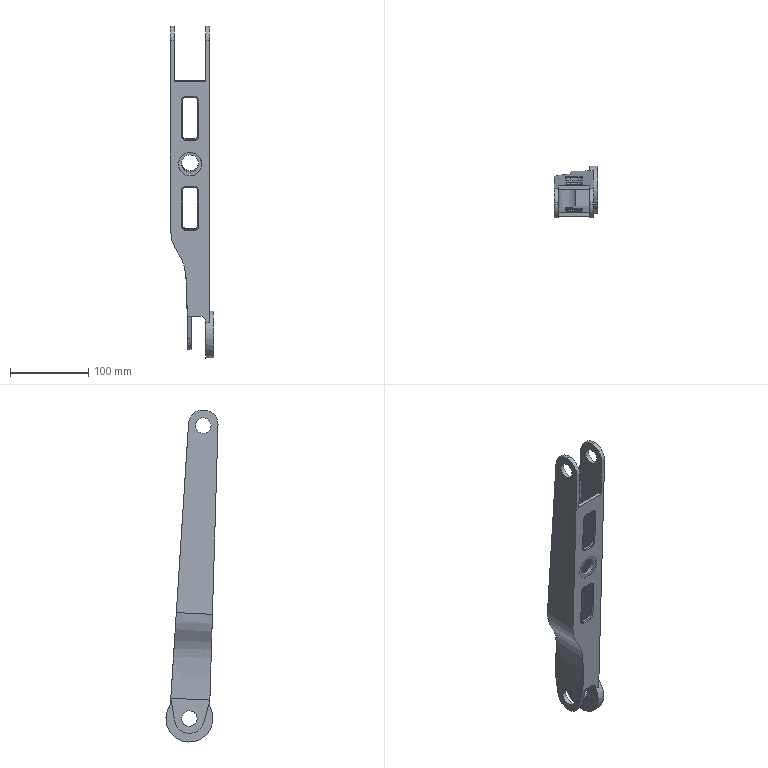Component | NX | CCJ-004 | 1 solid | 133 faces | volume 271570 mm3 | cylinder 62 | plane 37 | spline 33 | other 1 | commonest cylinder face diameters 2 x32 10 x16 20 x4 36 x4 22 x2 38.275 x1 16 x1 60 x1